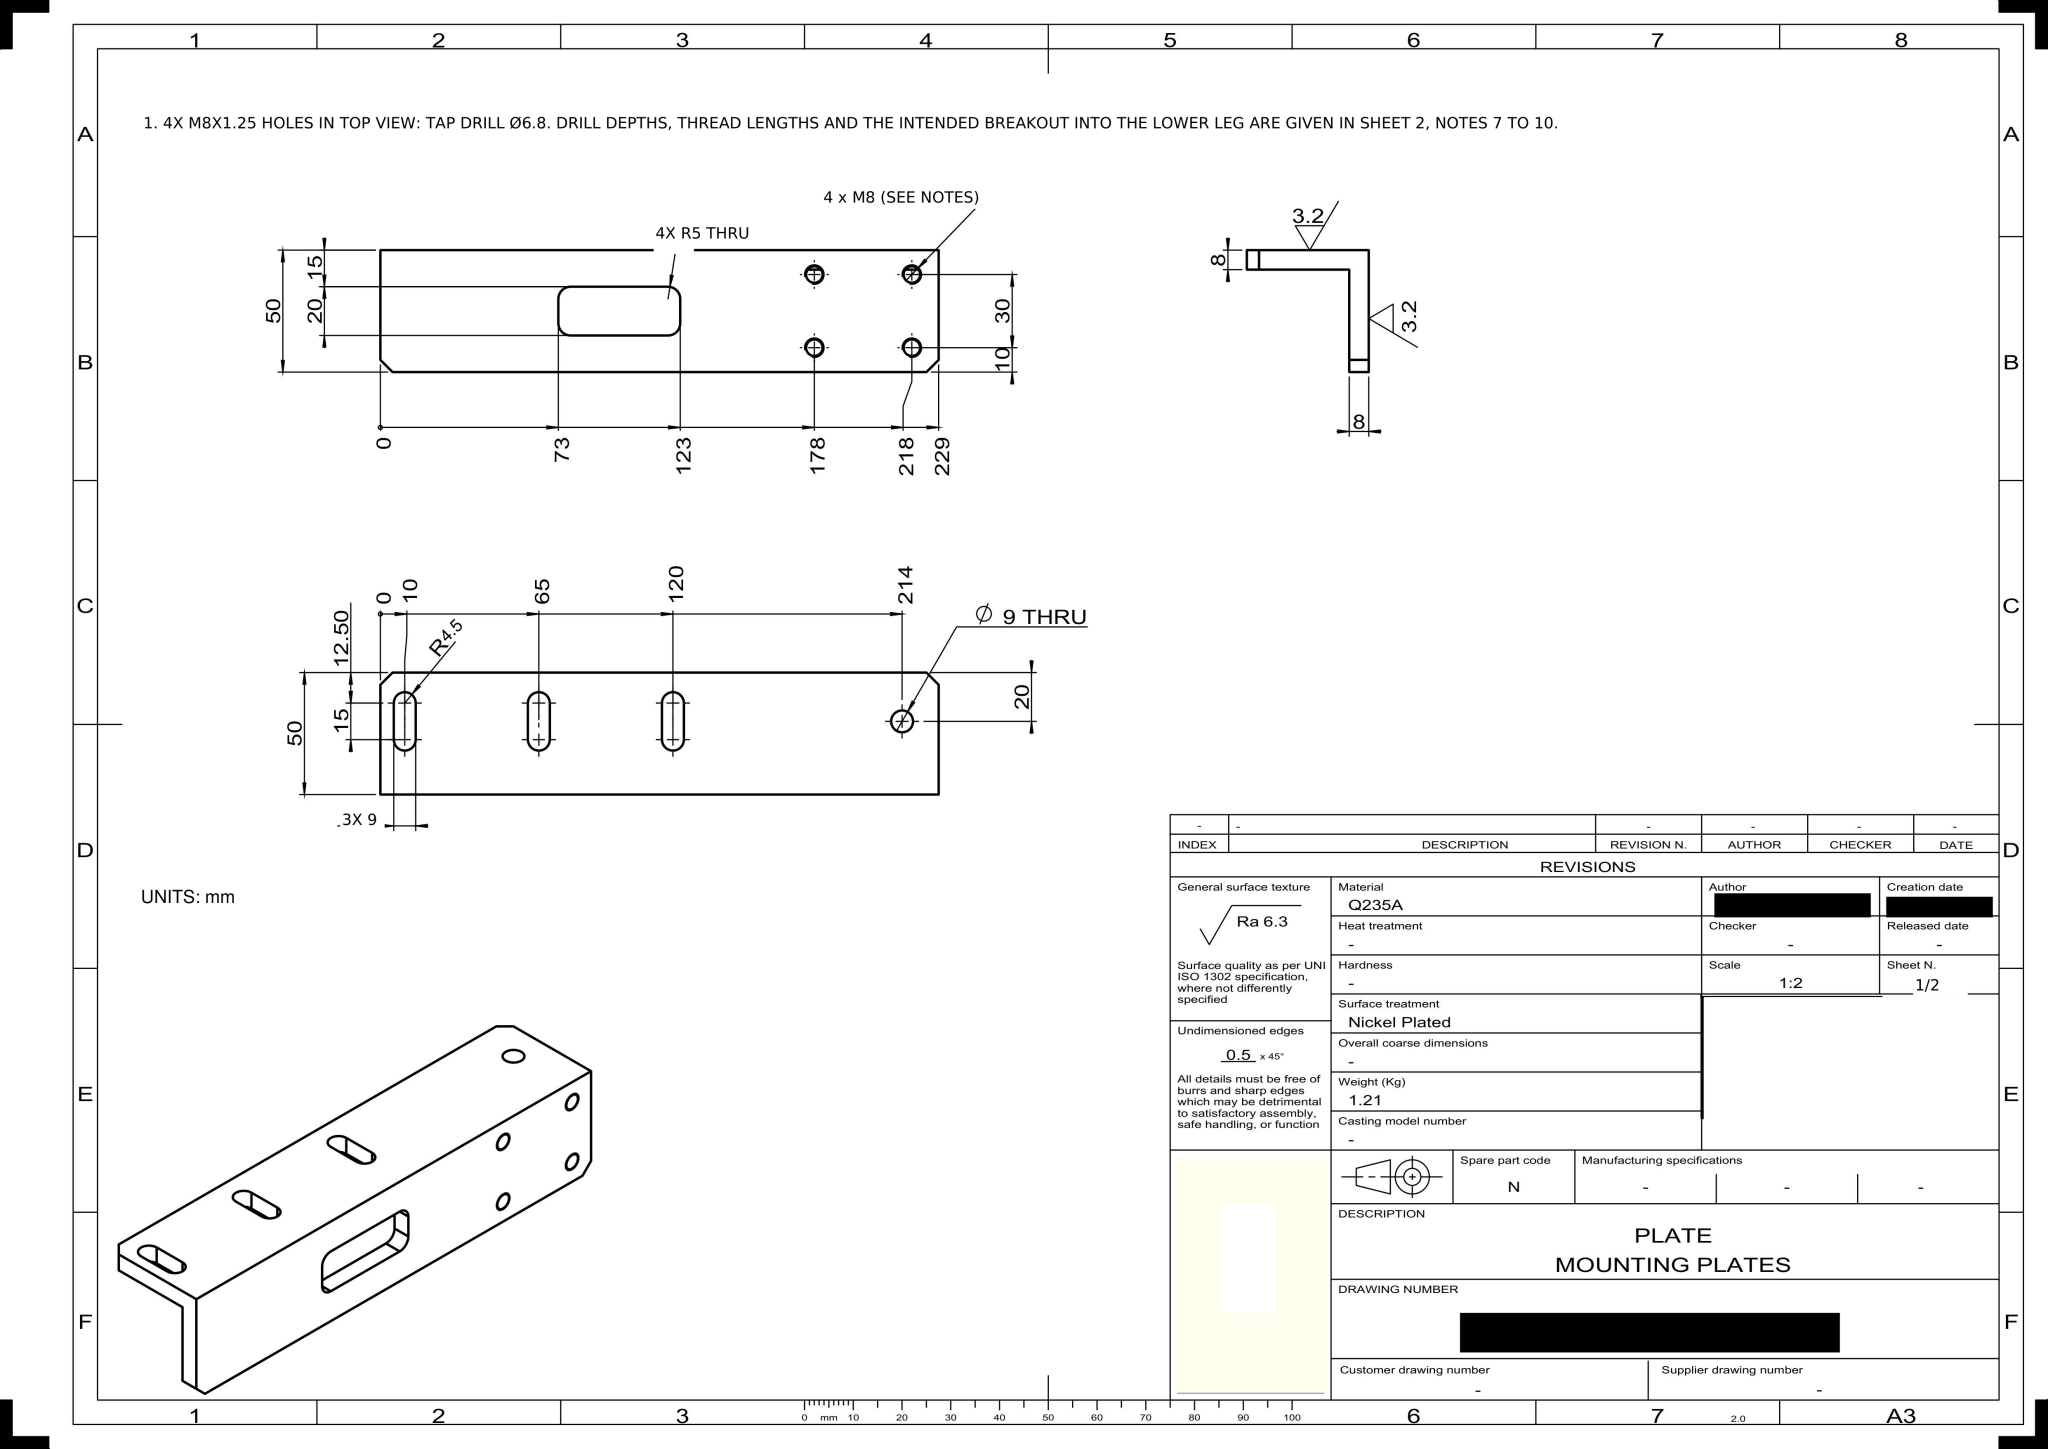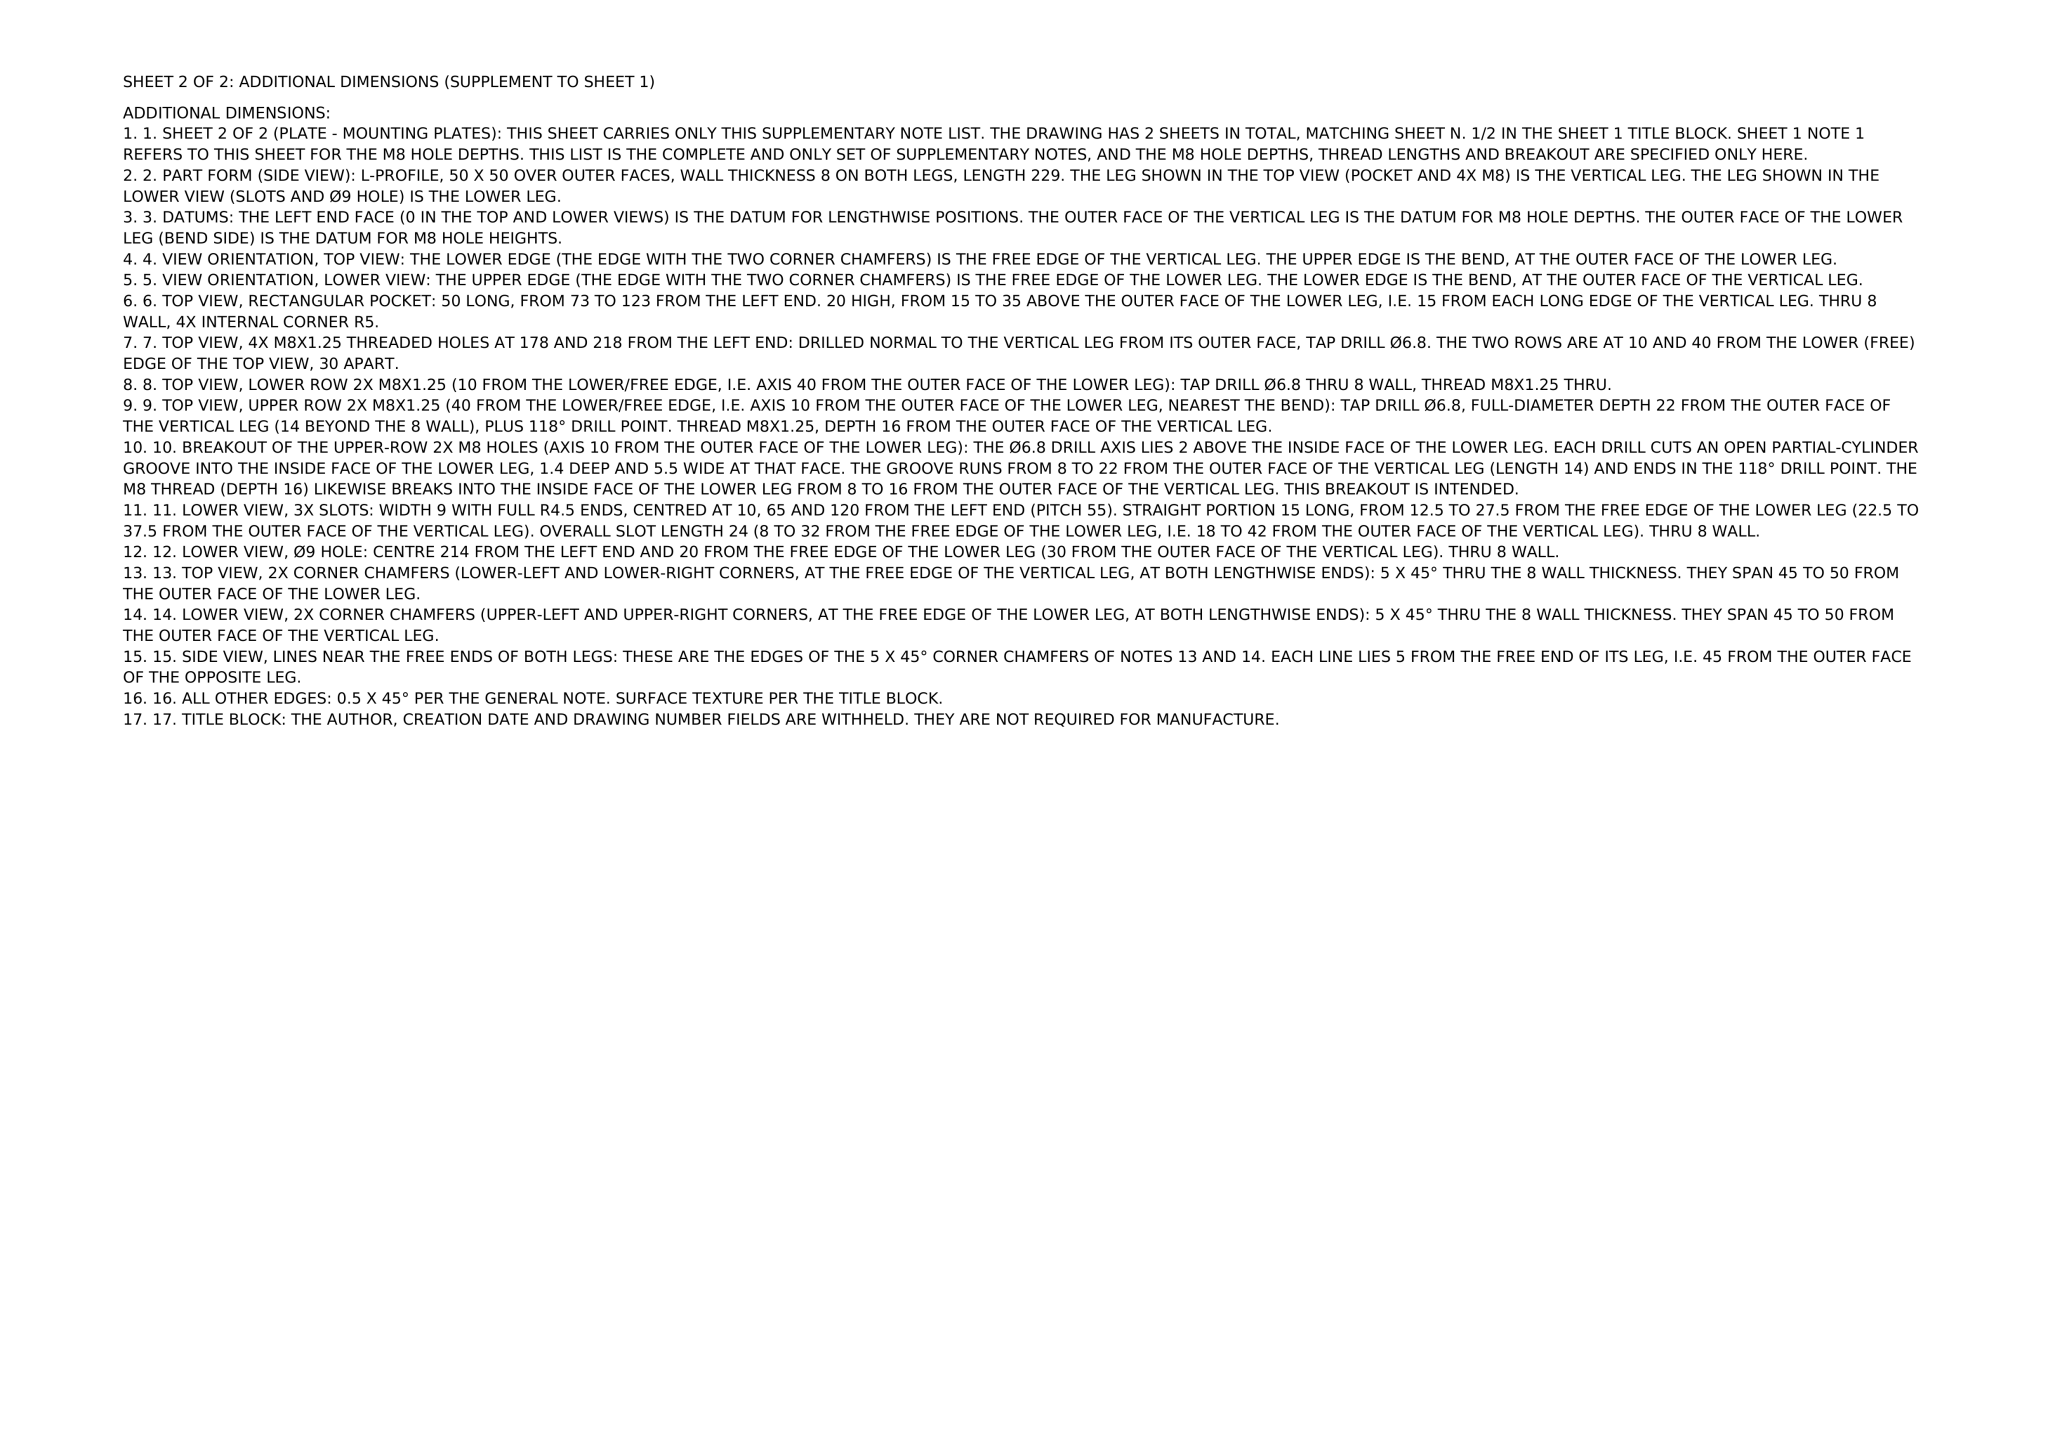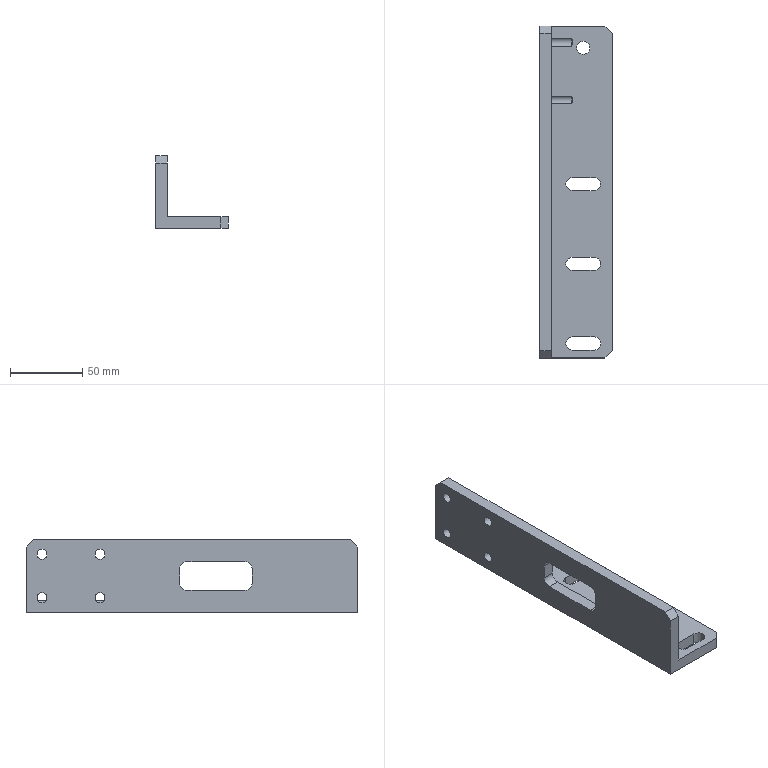Part | NX | mm | 1 solid | 39 faces | box 50 x 229 x 50 mm | volume 153723 mm3 | plane 22 | cylinder 15 | cone 2 | commonest cylinder face diameters 9 x7 6.8 x4 10 x4